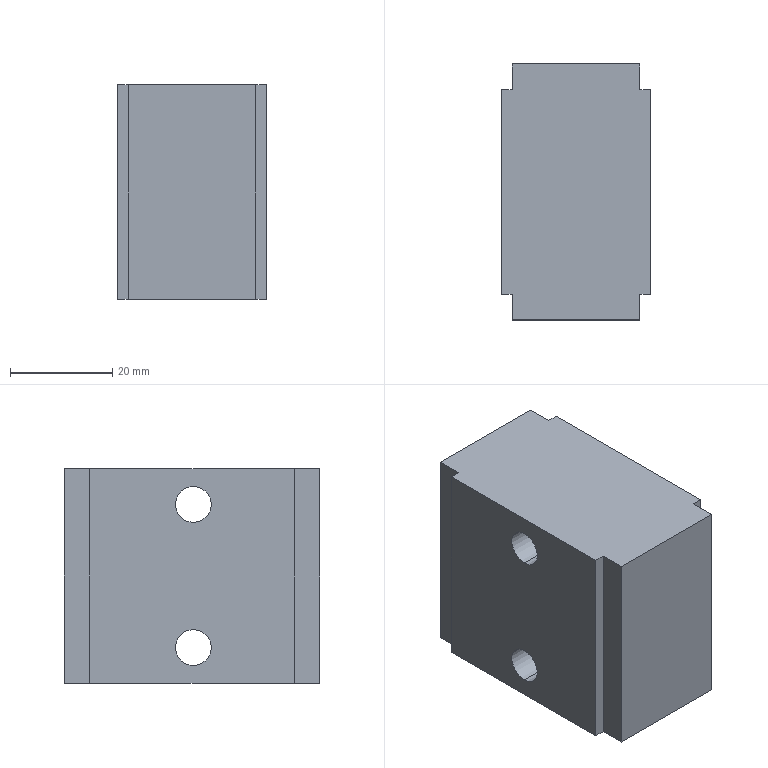Component | SolidWorks | SuctionCupMountingQuickConnector-1 | 1 solid | 18 faces | box 29 x 50 x 42 mm | volume 56988 mm3 | plane 14 | cylinder 4 | commonest cylinder face diameters 7 x4
build123d program:
from build123d import *

# Parameters (mm, degrees)
SKETCH2_W                = 25
SKETCH2_H                = 50
BOSS_EXTRUDE1_DEPTH      = 42
SKETCH3_W                = 2
SKETCH3_H                = 40
BOSS_EXTRUDE2_DEPTH      = 42
F_7_0_7_DIAMETER_HOLE1_D = 7


with BuildPart() as part:
    # Sketch2 → Boss-Extrude1 (new body)
    with BuildSketch(Plane.XY):
        with Locations((47.731, -80.656)):
            Rectangle(SKETCH2_W, SKETCH2_H)
    extrude(amount=-BOSS_EXTRUDE1_DEPTH)

    # Sketch3 → Boss-Extrude2 (add)
    with BuildSketch(Plane.XY):
        with Locations((34.231, -80.656)):
            Rectangle(SKETCH3_W, SKETCH3_H)
        with Locations((61.231, -80.656)):
            Rectangle(SKETCH3_W, SKETCH3_H)
    extrude(amount=-BOSS_EXTRUDE2_DEPTH)

    # 7.0 _7_ Diameter Hole1 (through all)
    with Locations(Plane(origin=(62.231, 0, 0), x_dir=(0, 0, -1), z_dir=(1, 0, 0))):
        with Locations((7, -80.906), (35, -80.906)):
            Hole(F_7_0_7_DIAMETER_HOLE1_D / 2)


solid = part.part

# Placed as in the assembly
solid = solid.moved(Location((-666.927, 2.005, 394.468), (0, 0, 0)))
STEP:
#1=COLOUR_RGB('',0.7922,0.8196,0.9333);
#2=FILL_AREA_STYLE_COLOUR('',#1);
#3=FILL_AREA_STYLE('',(#2));
#4=SURFACE_STYLE_FILL_AREA(#3);
#5=SURFACE_SIDE_STYLE('',(#4));
#6=SURFACE_STYLE_USAGE(.BOTH.,#5);
#7=PRESENTATION_STYLE_ASSIGNMENT((#6));
#8=CARTESIAN_POINT('',(-23.807,-3.106,14.014));
#9=VERTEX_POINT('',#8);
#10=CARTESIAN_POINT('',(-23.807,-3.106,14.29));
#11=VERTEX_POINT('',#10);
#12=CARTESIAN_POINT('',(-23.807,-3.106,14.152));
#13=DIRECTION('',(-1.,-0.,-0.));
#14=DIRECTION('',(0.,0.,1.));
#15=AXIS2_PLACEMENT_3D('',#12,#13,#14);
#16=CIRCLE('',#15,0.1378);
#17=EDGE_CURVE('',#9,#11,#16,.T.);
#18=ORIENTED_EDGE('',*,*,#17,.F.);
#19=CARTESIAN_POINT('',(-24.949,-3.106,14.014));
#20=VERTEX_POINT('',#19);
#21=CARTESIAN_POINT('',(-24.949,-3.106,14.014));
#22=DIRECTION('',(-1.,-0.,-0.));
#23=VECTOR('',#22,39.37);
#24=LINE('',#21,#23);
#25=EDGE_CURVE('',#9,#20,#24,.T.);
#26=ORIENTED_EDGE('',*,*,#25,.T.);
#27=CARTESIAN_POINT('',(-24.949,-3.106,14.29));
#28=VERTEX_POINT('',#27);
#29=CARTESIAN_POINT('',(-24.949,-3.106,14.152));
#30=DIRECTION('',(-1.,-0.,-0.));
#31=DIRECTION('',(0.,0.,1.));
#32=AXIS2_PLACEMENT_3D('',#29,#30,#31);
#33=CIRCLE('',#32,0.1378);
#34=EDGE_CURVE('',#20,#28,#33,.T.);
#35=ORIENTED_EDGE('',*,*,#34,.T.);
#36=CARTESIAN_POINT('',(-24.949,-3.106,14.29));
#37=DIRECTION('',(-1.,-0.,-0.));
#38=VECTOR('',#37,39.37);
#39=LINE('',#36,#38);
#40=EDGE_CURVE('',#11,#28,#39,.T.);
#41=ORIENTED_EDGE('',*,*,#40,.F.);
#42=EDGE_LOOP('',(#18,#26,#35,#41));
#43=FACE_OUTER_BOUND('',#42,.T.);
#44=CARTESIAN_POINT('',(-24.949,-3.106,14.152));
#45=DIRECTION('',(-1.,-0.,-0.));
#46=DIRECTION('',(0.,0.,1.));
#47=AXIS2_PLACEMENT_3D('',#44,#45,#46);
#48=CYLINDRICAL_SURFACE('',#47,0.1378);
#49=ADVANCED_FACE('',(#43),#48,.F.);
#50=CARTESIAN_POINT('',(-23.807,-3.106,15.117));
#51=VERTEX_POINT('',#50);
#52=CARTESIAN_POINT('',(-23.807,-3.106,15.392));
#53=VERTEX_POINT('',#52);
#54=CARTESIAN_POINT('',(-23.807,-3.106,15.255));
#55=DIRECTION('',(-1.,-0.,-0.));
#56=DIRECTION('',(0.,0.,1.));
#57=AXIS2_PLACEMENT_3D('',#54,#55,#56);
#58=CIRCLE('',#57,0.1378);
#59=EDGE_CURVE('',#51,#53,#58,.T.);
#60=ORIENTED_EDGE('',*,*,#59,.F.);
#61=CARTESIAN_POINT('',(-24.949,-3.106,15.117));
#62=VERTEX_POINT('',#61);
#63=CARTESIAN_POINT('',(-24.949,-3.106,15.117));
#64=DIRECTION('',(-1.,-0.,-0.));
#65=VECTOR('',#64,39.37);
#66=LINE('',#63,#65);
#67=EDGE_CURVE('',#51,#62,#66,.T.);
#68=ORIENTED_EDGE('',*,*,#67,.T.);
#69=CARTESIAN_POINT('',(-24.949,-3.106,15.392));
#70=VERTEX_POINT('',#69);
#71=CARTESIAN_POINT('',(-24.949,-3.106,15.255));
#72=DIRECTION('',(-1.,-0.,-0.));
#73=DIRECTION('',(0.,0.,1.));
#74=AXIS2_PLACEMENT_3D('',#71,#72,#73);
#75=CIRCLE('',#74,0.1378);
#76=EDGE_CURVE('',#62,#70,#75,.T.);
#77=ORIENTED_EDGE('',*,*,#76,.T.);
#78=CARTESIAN_POINT('',(-24.949,-3.106,15.392));
#79=DIRECTION('',(-1.,-0.,-0.));
#80=VECTOR('',#79,39.37);
#81=LINE('',#78,#80);
#82=EDGE_CURVE('',#53,#70,#81,.T.);
#83=ORIENTED_EDGE('',*,*,#82,.F.);
#84=EDGE_LOOP('',(#60,#68,#77,#83));
#85=FACE_OUTER_BOUND('',#84,.T.);
#86=CARTESIAN_POINT('',(-24.949,-3.106,15.255));
#87=DIRECTION('',(-1.,-0.,-0.));
#88=DIRECTION('',(0.,0.,1.));
#89=AXIS2_PLACEMENT_3D('',#86,#87,#88);
#90=CYLINDRICAL_SURFACE('',#89,0.1378);
#91=ADVANCED_FACE('',(#85),#90,.F.);
#92=CARTESIAN_POINT('',(-24.87,-4.081,15.53));
#93=VERTEX_POINT('',#92);
#94=CARTESIAN_POINT('',(-24.87,-3.884,15.53));
#95=VERTEX_POINT('',#94);
#96=CARTESIAN_POINT('',(-24.87,-2.112,15.53));
#97=DIRECTION('',(-0.,1.,-0.));
#98=VECTOR('',#97,39.37);
#99=LINE('',#96,#98);
#100=EDGE_CURVE('',#93,#95,#99,.T.);
#101=ORIENTED_EDGE('',*,*,#100,.T.);
#102=CARTESIAN_POINT('',(-24.87,-3.884,13.877));
#103=VERTEX_POINT('',#102);
#104=CARTESIAN_POINT('',(-24.87,-3.884,15.53));
#105=DIRECTION('',(0.,-0.,-1.));
#106=VECTOR('',#105,39.37);
#107=LINE('',#104,#106);
#108=EDGE_CURVE('',#95,#103,#107,.T.);
#109=ORIENTED_EDGE('',*,*,#108,.T.);
#110=CARTESIAN_POINT('',(-24.87,-4.081,13.877));
#111=VERTEX_POINT('',#110);
#112=CARTESIAN_POINT('',(-24.87,-2.112,13.877));
#113=DIRECTION('',(-0.,1.,-0.));
#114=VECTOR('',#113,39.37);
#115=LINE('',#112,#114);
#116=EDGE_CURVE('',#111,#103,#115,.T.);
#117=ORIENTED_EDGE('',*,*,#116,.F.);
#118=CARTESIAN_POINT('',(-24.87,-4.081,15.53));
#119=DIRECTION('',(0.,-0.,-1.));
#120=VECTOR('',#119,39.37);
#121=LINE('',#118,#120);
#122=EDGE_CURVE('',#93,#111,#121,.T.);
#123=ORIENTED_EDGE('',*,*,#122,.F.);
#124=EDGE_LOOP('',(#101,#109,#117,#123));
#125=FACE_OUTER_BOUND('',#124,.T.);
#126=CARTESIAN_POINT('',(-24.87,-2.112,15.53));
#127=DIRECTION('',(-1.,-0.,-0.));
#128=DIRECTION('',(-0.,1.,-0.));
#129=AXIS2_PLACEMENT_3D('',#126,#127,#128);
#130=PLANE('',#129);
#131=ADVANCED_FACE('',(#125),#130,.T.);
#132=CARTESIAN_POINT('',(-23.886,-2.112,15.53));
#133=VERTEX_POINT('',#132);
#134=CARTESIAN_POINT('',(-23.886,-2.309,15.53));
#135=VERTEX_POINT('',#134);
#136=CARTESIAN_POINT('',(-23.886,-2.112,15.53));
#137=DIRECTION('',(0.,-1.,0.));
#138=VECTOR('',#137,39.37);
#139=LINE('',#136,#138);
#140=EDGE_CURVE('',#133,#135,#139,.T.);
#141=ORIENTED_EDGE('',*,*,#140,.T.);
#142=CARTESIAN_POINT('',(-23.886,-2.309,13.877));
#143=VERTEX_POINT('',#142);
#144=CARTESIAN_POINT('',(-23.886,-2.309,15.53));
#145=DIRECTION('',(0.,-0.,-1.));
#146=VECTOR('',#145,39.37);
#147=LINE('',#144,#146);
#148=EDGE_CURVE('',#135,#143,#147,.T.);
#149=ORIENTED_EDGE('',*,*,#148,.T.);
#150=CARTESIAN_POINT('',(-23.886,-2.112,13.877));
#151=VERTEX_POINT('',#150);
#152=CARTESIAN_POINT('',(-23.886,-2.112,13.877));
#153=DIRECTION('',(0.,-1.,0.));
#154=VECTOR('',#153,39.37);
#155=LINE('',#152,#154);
#156=EDGE_CURVE('',#151,#143,#155,.T.);
#157=ORIENTED_EDGE('',*,*,#156,.F.);
#158=CARTESIAN_POINT('',(-23.886,-2.112,15.53));
#159=DIRECTION('',(0.,-0.,-1.));
#160=VECTOR('',#159,39.37);
#161=LINE('',#158,#160);
#162=EDGE_CURVE('',#133,#151,#161,.T.);
#163=ORIENTED_EDGE('',*,*,#162,.F.);
#164=EDGE_LOOP('',(#141,#149,#157,#163));
#165=FACE_OUTER_BOUND('',#164,.T.);
#166=CARTESIAN_POINT('',(-23.886,-2.112,15.53));
#167=DIRECTION('',(1.,0.,0.));
#168=DIRECTION('',(0.,-1.,0.));
#169=AXIS2_PLACEMENT_3D('',#166,#167,#168);
#170=PLANE('',#169);
#171=ADVANCED_FACE('',(#165),#170,.T.);
#172=CARTESIAN_POINT('',(-23.886,-3.884,15.53));
#173=VERTEX_POINT('',#172);
#174=CARTESIAN_POINT('',(-23.886,-3.884,13.877));
#175=VERTEX_POINT('',#174);
#176=CARTESIAN_POINT('',(-23.886,-3.884,15.53));
#177=DIRECTION('',(0.,-0.,-1.));
#178=VECTOR('',#177,39.37);
#179=LINE('',#176,#178);
#180=EDGE_CURVE('',#173,#175,#179,.T.);
#181=ORIENTED_EDGE('',*,*,#180,.F.);
#182=CARTESIAN_POINT('',(-23.886,-4.081,15.53));
#183=VERTEX_POINT('',#182);
#184=CARTESIAN_POINT('',(-23.886,-2.112,15.53));
#185=DIRECTION('',(0.,-1.,0.));
#186=VECTOR('',#185,39.37);
#187=LINE('',#184,#186);
#188=EDGE_CURVE('',#173,#183,#187,.T.);
#189=ORIENTED_EDGE('',*,*,#188,.T.);
#190=CARTESIAN_POINT('',(-23.886,-4.081,13.877));
#191=VERTEX_POINT('',#190);
#192=CARTESIAN_POINT('',(-23.886,-4.081,15.53));
#193=DIRECTION('',(0.,-0.,-1.));
#194=VECTOR('',#193,39.37);
#195=LINE('',#192,#194);
#196=EDGE_CURVE('',#183,#191,#195,.T.);
#197=ORIENTED_EDGE('',*,*,#196,.T.);
#198=CARTESIAN_POINT('',(-23.886,-2.112,13.877));
#199=DIRECTION('',(0.,-1.,0.));
#200=VECTOR('',#199,39.37);
#201=LINE('',#198,#200);
#202=EDGE_CURVE('',#175,#191,#201,.T.);
#203=ORIENTED_EDGE('',*,*,#202,.F.);
#204=EDGE_LOOP('',(#181,#189,#197,#203));
#205=FACE_OUTER_BOUND('',#204,.T.);
#206=CARTESIAN_POINT('',(-23.886,-2.112,15.53));
#207=DIRECTION('',(1.,0.,0.));
#208=DIRECTION('',(0.,-1.,0.));
#209=AXIS2_PLACEMENT_3D('',#206,#207,#208);
#210=PLANE('',#209);
#211=ADVANCED_FACE('',(#205),#210,.T.);
#212=CARTESIAN_POINT('',(-24.87,-2.112,13.877));
#213=VERTEX_POINT('',#212);
#214=CARTESIAN_POINT('',(-23.886,-2.112,13.877));
#215=DIRECTION('',(1.,0.,0.));
#216=VECTOR('',#215,39.37);
#217=LINE('',#214,#216);
#218=EDGE_CURVE('',#213,#151,#217,.T.);
#219=ORIENTED_EDGE('',*,*,#218,.F.);
#220=CARTESIAN_POINT('',(-24.87,-2.112,15.53));
#221=VERTEX_POINT('',#220);
#222=CARTESIAN_POINT('',(-24.87,-2.112,15.53));
#223=DIRECTION('',(0.,-0.,-1.));
#224=VECTOR('',#223,39.37);
#225=LINE('',#222,#224);
#226=EDGE_CURVE('',#221,#213,#225,.T.);
#227=ORIENTED_EDGE('',*,*,#226,.F.);
#228=CARTESIAN_POINT('',(-23.886,-2.112,15.53));
#229=DIRECTION('',(1.,0.,0.));
#230=VECTOR('',#229,39.37);
#231=LINE('',#228,#230);
#232=EDGE_CURVE('',#221,#133,#231,.T.);
#233=ORIENTED_EDGE('',*,*,#232,.T.);
#234=ORIENTED_EDGE('',*,*,#162,.T.);
#235=EDGE_LOOP('',(#219,#227,#233,#234));
#236=FACE_OUTER_BOUND('',#235,.T.);
#237=CARTESIAN_POINT('',(-23.886,-2.112,15.53));
#238=DIRECTION('',(0.,1.,-0.));
#239=DIRECTION('',(0.,-0.,-1.));
#240=AXIS2_PLACEMENT_3D('',#237,#238,#239);
#241=PLANE('',#240);
#242=ADVANCED_FACE('',(#236),#241,.T.);
#243=CARTESIAN_POINT('',(-24.87,-2.309,15.53));
#244=VERTEX_POINT('',#243);
#245=CARTESIAN_POINT('',(-24.87,-2.309,13.877));
#246=VERTEX_POINT('',#245);
#247=CARTESIAN_POINT('',(-24.87,-2.309,15.53));
#248=DIRECTION('',(0.,-0.,-1.));
#249=VECTOR('',#248,39.37);
#250=LINE('',#247,#249);
#251=EDGE_CURVE('',#244,#246,#250,.T.);
#252=ORIENTED_EDGE('',*,*,#251,.F.);
#253=CARTESIAN_POINT('',(-24.87,-2.112,15.53));
#254=DIRECTION('',(-0.,1.,-0.));
#255=VECTOR('',#254,39.37);
#256=LINE('',#253,#255);
#257=EDGE_CURVE('',#244,#221,#256,.T.);
#258=ORIENTED_EDGE('',*,*,#257,.T.);
#259=ORIENTED_EDGE('',*,*,#226,.T.);
#260=CARTESIAN_POINT('',(-24.87,-2.112,13.877));
#261=DIRECTION('',(-0.,1.,-0.));
#262=VECTOR('',#261,39.37);
#263=LINE('',#260,#262);
#264=EDGE_CURVE('',#246,#213,#263,.T.);
#265=ORIENTED_EDGE('',*,*,#264,.F.);
#266=EDGE_LOOP('',(#252,#258,#259,#265));
#267=FACE_OUTER_BOUND('',#266,.T.);
#268=CARTESIAN_POINT('',(-24.87,-2.112,15.53));
#269=DIRECTION('',(-1.,-0.,-0.));
#270=DIRECTION('',(-0.,1.,-0.));
#271=AXIS2_PLACEMENT_3D('',#268,#269,#270);
#272=PLANE('',#271);
#273=ADVANCED_FACE('',(#267),#272,.T.);
#274=CARTESIAN_POINT('',(-23.886,-4.081,13.877));
#275=DIRECTION('',(-1.,-0.,-0.));
#276=VECTOR('',#275,39.37);
#277=LINE('',#274,#276);
#278=EDGE_CURVE('',#191,#111,#277,.T.);
#279=ORIENTED_EDGE('',*,*,#278,.F.);
#280=ORIENTED_EDGE('',*,*,#196,.F.);
#281=CARTESIAN_POINT('',(-23.886,-4.081,15.53));
#282=DIRECTION('',(-1.,-0.,-0.));
#283=VECTOR('',#282,39.37);
#284=LINE('',#281,#283);
#285=EDGE_CURVE('',#183,#93,#284,.T.);
#286=ORIENTED_EDGE('',*,*,#285,.T.);
#287=ORIENTED_EDGE('',*,*,#122,.T.);
#288=EDGE_LOOP('',(#279,#280,#286,#287));
#289=FACE_OUTER_BOUND('',#288,.T.);
#290=CARTESIAN_POINT('',(-23.886,-4.081,15.53));
#291=DIRECTION('',(0.,-1.,0.));
#292=DIRECTION('',(-0.,0.,1.));
#293=AXIS2_PLACEMENT_3D('',#290,#291,#292);
#294=PLANE('',#293);
#295=ADVANCED_FACE('',(#289),#294,.T.);
#296=ORIENTED_EDGE('',*,*,#140,.F.);
#297=ORIENTED_EDGE('',*,*,#232,.F.);
#298=ORIENTED_EDGE('',*,*,#257,.F.);
#299=CARTESIAN_POINT('',(-24.949,-2.309,15.53));
#300=VERTEX_POINT('',#299);
#301=CARTESIAN_POINT('',(-22.499,-2.309,15.53));
#302=DIRECTION('',(-1.,-0.,-0.));
#303=VECTOR('',#302,39.37);
#304=LINE('',#301,#303);
#305=EDGE_CURVE('',#244,#300,#304,.T.);
#306=ORIENTED_EDGE('',*,*,#305,.T.);
#307=CARTESIAN_POINT('',(-24.949,-3.884,15.53));
#308=VERTEX_POINT('',#307);
#309=CARTESIAN_POINT('',(-24.949,0.07892,15.53));
#310=DIRECTION('',(0.,-1.,0.));
#311=VECTOR('',#310,39.37);
#312=LINE('',#309,#311);
#313=EDGE_CURVE('',#300,#308,#312,.T.);
#314=ORIENTED_EDGE('',*,*,#313,.T.);
#315=CARTESIAN_POINT('',(-22.499,-3.884,15.53));
#316=DIRECTION('',(-1.,-0.,-0.));
#317=VECTOR('',#316,39.37);
#318=LINE('',#315,#317);
#319=EDGE_CURVE('',#95,#308,#318,.T.);
#320=ORIENTED_EDGE('',*,*,#319,.F.);
#321=ORIENTED_EDGE('',*,*,#100,.F.);
#322=ORIENTED_EDGE('',*,*,#285,.F.);
#323=ORIENTED_EDGE('',*,*,#188,.F.);
#324=CARTESIAN_POINT('',(-23.807,-3.884,15.53));
#325=VERTEX_POINT('',#324);
#326=CARTESIAN_POINT('',(-22.499,-3.884,15.53));
#327=DIRECTION('',(-1.,-0.,-0.));
#328=VECTOR('',#327,39.37);
#329=LINE('',#326,#328);
#330=EDGE_CURVE('',#325,#173,#329,.T.);
#331=ORIENTED_EDGE('',*,*,#330,.F.);
#332=CARTESIAN_POINT('',(-23.807,-2.309,15.53));
#333=VERTEX_POINT('',#332);
#334=CARTESIAN_POINT('',(-23.807,0.07892,15.53));
#335=DIRECTION('',(0.,-1.,0.));
#336=VECTOR('',#335,39.37);
#337=LINE('',#334,#336);
#338=EDGE_CURVE('',#333,#325,#337,.T.);
#339=ORIENTED_EDGE('',*,*,#338,.F.);
#340=CARTESIAN_POINT('',(-22.499,-2.309,15.53));
#341=DIRECTION('',(-1.,-0.,-0.));
#342=VECTOR('',#341,39.37);
#343=LINE('',#340,#342);
#344=EDGE_CURVE('',#333,#135,#343,.T.);
#345=ORIENTED_EDGE('',*,*,#344,.T.);
#346=EDGE_LOOP('',(#296,#297,#298,#306,#314,#320,#321,#322,#323,#331,#339,#345));
#347=FACE_OUTER_BOUND('',#346,.T.);
#348=CARTESIAN_POINT('',(-22.499,0.07892,15.53));
#349=DIRECTION('',(0.,-0.,-1.));
#350=DIRECTION('',(-1.,-0.,-0.));
#351=AXIS2_PLACEMENT_3D('',#348,#349,#350);
#352=PLANE('',#351);
#353=ADVANCED_FACE('',(#347),#352,.F.);
#354=ORIENTED_EDGE('',*,*,#156,.T.);
#355=CARTESIAN_POINT('',(-23.807,-2.309,13.877));
#356=VERTEX_POINT('',#355);
#357=CARTESIAN_POINT('',(-22.499,-2.309,13.877));
#358=DIRECTION('',(-1.,-0.,-0.));
#359=VECTOR('',#358,39.37);
#360=LINE('',#357,#359);
#361=EDGE_CURVE('',#356,#143,#360,.T.);
#362=ORIENTED_EDGE('',*,*,#361,.F.);
#363=CARTESIAN_POINT('',(-23.807,-3.884,13.877));
#364=VERTEX_POINT('',#363);
#365=CARTESIAN_POINT('',(-23.807,0.07892,13.877));
#366=DIRECTION('',(0.,-1.,0.));
#367=VECTOR('',#366,39.37);
#368=LINE('',#365,#367);
#369=EDGE_CURVE('',#356,#364,#368,.T.);
#370=ORIENTED_EDGE('',*,*,#369,.T.);
#371=CARTESIAN_POINT('',(-22.499,-3.884,13.877));
#372=DIRECTION('',(-1.,-0.,-0.));
#373=VECTOR('',#372,39.37);
#374=LINE('',#371,#373);
#375=EDGE_CURVE('',#364,#175,#374,.T.);
#376=ORIENTED_EDGE('',*,*,#375,.T.);
#377=ORIENTED_EDGE('',*,*,#202,.T.);
#378=ORIENTED_EDGE('',*,*,#278,.T.);
#379=ORIENTED_EDGE('',*,*,#116,.T.);
#380=CARTESIAN_POINT('',(-24.949,-3.884,13.877));
#381=VERTEX_POINT('',#380);
#382=CARTESIAN_POINT('',(-22.499,-3.884,13.877));
#383=DIRECTION('',(-1.,-0.,-0.));
#384=VECTOR('',#383,39.37);
#385=LINE('',#382,#384);
#386=EDGE_CURVE('',#103,#381,#385,.T.);
#387=ORIENTED_EDGE('',*,*,#386,.T.);
#388=CARTESIAN_POINT('',(-24.949,-2.309,13.877));
#389=VERTEX_POINT('',#388);
#390=CARTESIAN_POINT('',(-24.949,0.07892,13.877));
#391=DIRECTION('',(0.,-1.,0.));
#392=VECTOR('',#391,39.37);
#393=LINE('',#390,#392);
#394=EDGE_CURVE('',#389,#381,#393,.T.);
#395=ORIENTED_EDGE('',*,*,#394,.F.);
#396=CARTESIAN_POINT('',(-22.499,-2.309,13.877));
#397=DIRECTION('',(-1.,-0.,-0.));
#398=VECTOR('',#397,39.37);
#399=LINE('',#396,#398);
#400=EDGE_CURVE('',#246,#389,#399,.T.);
#401=ORIENTED_EDGE('',*,*,#400,.F.);
#402=ORIENTED_EDGE('',*,*,#264,.T.);
#403=ORIENTED_EDGE('',*,*,#218,.T.);
#404=EDGE_LOOP('',(#354,#362,#370,#376,#377,#378,#379,#387,#395,#401,#402,#403));
#405=FACE_OUTER_BOUND('',#404,.T.);
#406=CARTESIAN_POINT('',(-22.499,0.07892,13.877));
#407=DIRECTION('',(0.,-0.,-1.));
#408=DIRECTION('',(-1.,-0.,-0.));
#409=AXIS2_PLACEMENT_3D('',#406,#407,#408);
#410=PLANE('',#409);
#411=ADVANCED_FACE('',(#405),#410,.T.);
#412=CARTESIAN_POINT('',(-23.807,-3.106,14.152));
#413=DIRECTION('',(-1.,-0.,-0.));
#414=DIRECTION('',(0.,0.,1.));
#415=AXIS2_PLACEMENT_3D('',#412,#413,#414);
#416=CIRCLE('',#415,0.1378);
#417=EDGE_CURVE('',#11,#9,#416,.T.);
#418=ORIENTED_EDGE('',*,*,#417,.T.);
#419=ORIENTED_EDGE('',*,*,#17,.T.);
#420=EDGE_LOOP('',(#418,#419));
#421=FACE_BOUND('',#420,.T.);
#422=CARTESIAN_POINT('',(-23.807,-3.106,15.255));
#423=DIRECTION('',(-1.,-0.,-0.));
#424=DIRECTION('',(0.,0.,1.));
#425=AXIS2_PLACEMENT_3D('',#422,#423,#424);
#426=CIRCLE('',#425,0.1378);
#427=EDGE_CURVE('',#53,#51,#426,.T.);
#428=ORIENTED_EDGE('',*,*,#427,.T.);
#429=ORIENTED_EDGE('',*,*,#59,.T.);
#430=EDGE_LOOP('',(#428,#429));
#431=FACE_BOUND('',#430,.T.);
#432=ORIENTED_EDGE('',*,*,#369,.F.);
#433=CARTESIAN_POINT('',(-23.807,-2.309,15.53));
#434=DIRECTION('',(0.,-0.,-1.));
#435=VECTOR('',#434,39.37);
#436=LINE('',#433,#435);
#437=EDGE_CURVE('',#333,#356,#436,.T.);
#438=ORIENTED_EDGE('',*,*,#437,.F.);
#439=ORIENTED_EDGE('',*,*,#338,.T.);
#440=CARTESIAN_POINT('',(-23.807,-3.884,15.53));
#441=DIRECTION('',(0.,-0.,-1.));
#442=VECTOR('',#441,39.37);
#443=LINE('',#440,#442);
#444=EDGE_CURVE('',#325,#364,#443,.T.);
#445=ORIENTED_EDGE('',*,*,#444,.T.);
#446=EDGE_LOOP('',(#432,#438,#439,#445));
#447=FACE_OUTER_BOUND('',#446,.T.);
#448=CARTESIAN_POINT('',(-23.807,0.07892,15.53));
#449=DIRECTION('',(1.,0.,0.));
#450=DIRECTION('',(0.,-0.,-1.));
#451=AXIS2_PLACEMENT_3D('',#448,#449,#450);
#452=PLANE('',#451);
#453=ADVANCED_FACE('',(#421,#431,#447),#452,.T.);
#454=ORIENTED_EDGE('',*,*,#361,.T.);
#455=ORIENTED_EDGE('',*,*,#148,.F.);
#456=ORIENTED_EDGE('',*,*,#344,.F.);
#457=ORIENTED_EDGE('',*,*,#437,.T.);
#458=EDGE_LOOP('',(#454,#455,#456,#457));
#459=FACE_OUTER_BOUND('',#458,.T.);
#460=CARTESIAN_POINT('',(-22.499,-2.309,15.53));
#461=DIRECTION('',(0.,-1.,0.));
#462=DIRECTION('',(-0.,0.,1.));
#463=AXIS2_PLACEMENT_3D('',#460,#461,#462);
#464=PLANE('',#463);
#465=ADVANCED_FACE('',(#459),#464,.F.);
#466=ORIENTED_EDGE('',*,*,#375,.F.);
#467=ORIENTED_EDGE('',*,*,#444,.F.);
#468=ORIENTED_EDGE('',*,*,#330,.T.);
#469=ORIENTED_EDGE('',*,*,#180,.T.);
#470=EDGE_LOOP('',(#466,#467,#468,#469));
#471=FACE_OUTER_BOUND('',#470,.T.);
#472=CARTESIAN_POINT('',(-22.499,-3.884,15.53));
#473=DIRECTION('',(0.,-1.,0.));
#474=DIRECTION('',(-0.,0.,1.));
#475=AXIS2_PLACEMENT_3D('',#472,#473,#474);
#476=PLANE('',#475);
#477=ADVANCED_FACE('',(#471),#476,.T.);
#478=CARTESIAN_POINT('',(-24.949,-3.106,14.152));
#479=DIRECTION('',(-1.,-0.,-0.));
#480=DIRECTION('',(0.,0.,1.));
#481=AXIS2_PLACEMENT_3D('',#478,#479,#480);
#482=CIRCLE('',#481,0.1378);
#483=EDGE_CURVE('',#28,#20,#482,.T.);
#484=ORIENTED_EDGE('',*,*,#483,.F.);
#485=ORIENTED_EDGE('',*,*,#34,.F.);
#486=EDGE_LOOP('',(#484,#485));
#487=FACE_BOUND('',#486,.T.);
#488=CARTESIAN_POINT('',(-24.949,-3.106,15.255));
#489=DIRECTION('',(-1.,-0.,-0.));
#490=DIRECTION('',(0.,0.,1.));
#491=AXIS2_PLACEMENT_3D('',#488,#489,#490);
#492=CIRCLE('',#491,0.1378);
#493=EDGE_CURVE('',#70,#62,#492,.T.);
#494=ORIENTED_EDGE('',*,*,#493,.F.);
#495=ORIENTED_EDGE('',*,*,#76,.F.);
#496=EDGE_LOOP('',(#494,#495));
#497=FACE_BOUND('',#496,.T.);
#498=ORIENTED_EDGE('',*,*,#394,.T.);
#499=CARTESIAN_POINT('',(-24.949,-3.884,15.53));
#500=DIRECTION('',(0.,-0.,-1.));
#501=VECTOR('',#500,39.37);
#502=LINE('',#499,#501);
#503=EDGE_CURVE('',#308,#381,#502,.T.);
#504=ORIENTED_EDGE('',*,*,#503,.F.);
#505=ORIENTED_EDGE('',*,*,#313,.F.);
#506=CARTESIAN_POINT('',(-24.949,-2.309,15.53));
#507=DIRECTION('',(0.,-0.,-1.));
#508=VECTOR('',#507,39.37);
#509=LINE('',#506,#508);
#510=EDGE_CURVE('',#300,#389,#509,.T.);
#511=ORIENTED_EDGE('',*,*,#510,.T.);
#512=EDGE_LOOP('',(#498,#504,#505,#511));
#513=FACE_OUTER_BOUND('',#512,.T.);
#514=CARTESIAN_POINT('',(-24.949,0.07892,15.53));
#515=DIRECTION('',(1.,0.,0.));
#516=DIRECTION('',(0.,-0.,-1.));
#517=AXIS2_PLACEMENT_3D('',#514,#515,#516);
#518=PLANE('',#517);
#519=ADVANCED_FACE('',(#487,#497,#513),#518,.F.);
#520=ORIENTED_EDGE('',*,*,#386,.F.);
#521=ORIENTED_EDGE('',*,*,#108,.F.);
#522=ORIENTED_EDGE('',*,*,#319,.T.);
#523=ORIENTED_EDGE('',*,*,#503,.T.);
#524=EDGE_LOOP('',(#520,#521,#522,#523));
#525=FACE_OUTER_BOUND('',#524,.T.);
#526=CARTESIAN_POINT('',(-22.499,-3.884,15.53));
#527=DIRECTION('',(0.,-1.,0.));
#528=DIRECTION('',(-0.,0.,1.));
#529=AXIS2_PLACEMENT_3D('',#526,#527,#528);
#530=PLANE('',#529);
#531=ADVANCED_FACE('',(#525),#530,.T.);
#532=ORIENTED_EDGE('',*,*,#400,.T.);
#533=ORIENTED_EDGE('',*,*,#510,.F.);
#534=ORIENTED_EDGE('',*,*,#305,.F.);
#535=ORIENTED_EDGE('',*,*,#251,.T.);
#536=EDGE_LOOP('',(#532,#533,#534,#535));
#537=FACE_OUTER_BOUND('',#536,.T.);
#538=CARTESIAN_POINT('',(-22.499,-2.309,15.53));
#539=DIRECTION('',(0.,-1.,0.));
#540=DIRECTION('',(-0.,0.,1.));
#541=AXIS2_PLACEMENT_3D('',#538,#539,#540);
#542=PLANE('',#541);
#543=ADVANCED_FACE('',(#537),#542,.F.);
#544=ORIENTED_EDGE('',*,*,#67,.F.);
#545=ORIENTED_EDGE('',*,*,#427,.F.);
#546=ORIENTED_EDGE('',*,*,#82,.T.);
#547=ORIENTED_EDGE('',*,*,#493,.T.);
#548=EDGE_LOOP('',(#544,#545,#546,#547));
#549=FACE_OUTER_BOUND('',#548,.T.);
#550=CARTESIAN_POINT('',(-24.949,-3.106,15.255));
#551=DIRECTION('',(-1.,-0.,-0.));
#552=DIRECTION('',(0.,0.,1.));
#553=AXIS2_PLACEMENT_3D('',#550,#551,#552);
#554=CYLINDRICAL_SURFACE('',#553,0.1378);
#555=ADVANCED_FACE('',(#549),#554,.F.);
#556=ORIENTED_EDGE('',*,*,#25,.F.);
#557=ORIENTED_EDGE('',*,*,#417,.F.);
#558=ORIENTED_EDGE('',*,*,#40,.T.);
#559=ORIENTED_EDGE('',*,*,#483,.T.);
#560=EDGE_LOOP('',(#556,#557,#558,#559));
#561=FACE_OUTER_BOUND('',#560,.T.);
#562=CARTESIAN_POINT('',(-24.949,-3.106,14.152));
#563=DIRECTION('',(-1.,-0.,-0.));
#564=DIRECTION('',(0.,0.,1.));
#565=AXIS2_PLACEMENT_3D('',#562,#563,#564);
#566=CYLINDRICAL_SURFACE('',#565,0.1378);
#567=ADVANCED_FACE('',(#561),#566,.F.);
#568=CLOSED_SHELL('',(#49,#91,#131,#171,#211,#242,#273,#295,#353,#411,#453,#465,#477,#519,#531,#543,#555,#567));
#569=MANIFOLD_SOLID_BREP('',#568);
#570=STYLED_ITEM('',(#7),#569);
#571=(LENGTH_UNIT()NAMED_UNIT(*)SI_UNIT($,.METRE.));
#572=LENGTH_MEASURE_WITH_UNIT(LENGTH_MEASURE(0.0254),#571);
#573=DIMENSIONAL_EXPONENTS(1.,0.,0.,0.,0.,0.,0.);
#574=(CONVERSION_BASED_UNIT('',#572)LENGTH_UNIT()NAMED_UNIT(#573));
#575=UNCERTAINTY_MEASURE_WITH_UNIT(LENGTH_MEASURE(0.00001),#574,'','');
#576=(NAMED_UNIT(*)PLANE_ANGLE_UNIT()SI_UNIT($,.RADIAN.));
#577=(NAMED_UNIT(*)SI_UNIT($,.STERADIAN.)SOLID_ANGLE_UNIT());
#578=(GEOMETRIC_REPRESENTATION_CONTEXT(3)GLOBAL_UNCERTAINTY_ASSIGNED_CONTEXT((#575))GLOBAL_UNIT_ASSIGNED_CONTEXT((#574,#576,#577))REPRESENTATION_CONTEXT('',''));
#579=MECHANICAL_DESIGN_GEOMETRIC_PRESENTATION_REPRESENTATION('',(#570),#578);
#580=CARTESIAN_POINT('',(0.,0.,0.));
#581=DIRECTION('',(0.,0.,1.));
#582=DIRECTION('',(1.,0.,0.));
#583=AXIS2_PLACEMENT_3D('',#580,#581,#582);
#584=(LENGTH_UNIT()NAMED_UNIT(*)SI_UNIT($,.METRE.));
#585=LENGTH_MEASURE_WITH_UNIT(LENGTH_MEASURE(0.0254),#584);
#586=DIMENSIONAL_EXPONENTS(1.,0.,0.,0.,0.,0.,0.);
#587=(CONVERSION_BASED_UNIT('',#585)LENGTH_UNIT()NAMED_UNIT(#586));
#588=UNCERTAINTY_MEASURE_WITH_UNIT(LENGTH_MEASURE(0.00001),#587,'','');
#589=(NAMED_UNIT(*)PLANE_ANGLE_UNIT()SI_UNIT($,.RADIAN.));
#590=(NAMED_UNIT(*)SI_UNIT($,.STERADIAN.)SOLID_ANGLE_UNIT());
#591=(GEOMETRIC_REPRESENTATION_CONTEXT(3)GLOBAL_UNCERTAINTY_ASSIGNED_CONTEXT((#588))GLOBAL_UNIT_ASSIGNED_CONTEXT((#587,#589,#590))REPRESENTATION_CONTEXT('',''));
#592=ADVANCED_BREP_SHAPE_REPRESENTATION('',(#569,#583),#591);
#593=PRESENTATION_LAYER_ASSIGNMENT('','',(#570));